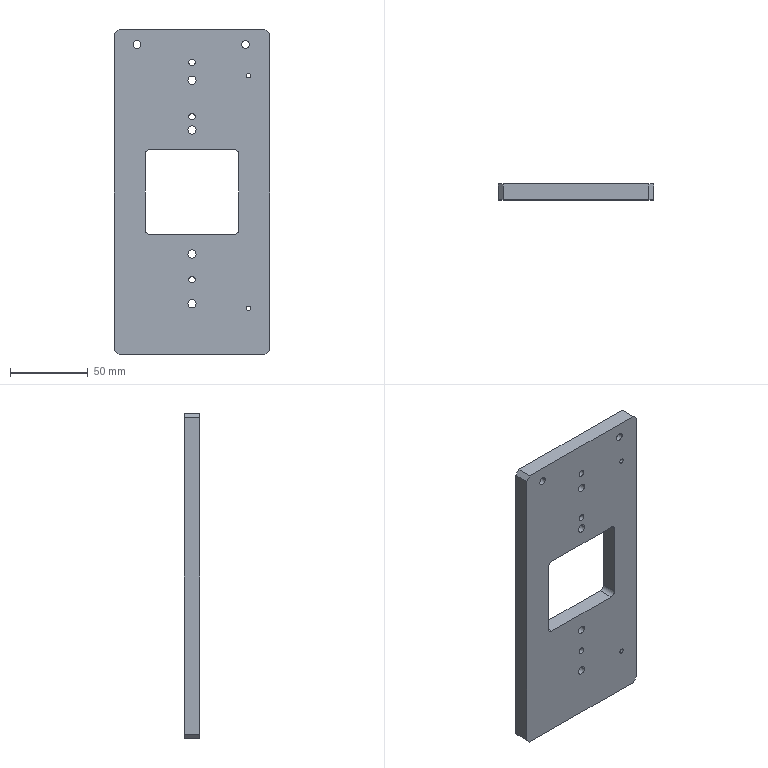Component | SolidWorks | SFTJ-06-CylinderBackPlate-1 | 1 solid | 60 faces | box 100 x 10 x 210 mm | volume 173599 mm3 | cylinder 38 | plane 18 | cone 4 | commonest cylinder face diameters 10 x8 5.3 x8 4.2 x6 5 x4 3.3 x4 3 x4 6 x4 | material 6061 Alloy
build123d program:
from build123d import *

# Parameters (mm, degrees)
SKETCH1_W                                            = 100
SKETCH1_H                                            = 210
BOSS_EXTRUDE1_DEPTH                                  = 5
CHAMFER1_SIZE                                        = 3
SKETCH2_W                                            = 60
SKETCH2_H                                            = 55
CUT_EXTRUDE1_DEPTH                                   = 117.726
FILLET1_R                                            = 3
M5_TAPPED_HOLE1_D                                    = 4.2
HOLE_SIZE_ACCORDING_TO_HEX_SOCKET_HEAD_C_D           = 5.3
HOLE_SIZE_ACCORDING_TO_HEX_SOCKET_HEAD_C_CBORE_D     = 10
HOLE_SIZE_ACCORDING_TO_HEX_SOCKET_HEAD_C_CBORE_DEPTH = 5.7
SIZE_MM_DOWEL_PIN_HOLE2_D                            = 3
M4_TAPPED_HOLE1_D                                    = 3.3
M4_TAPPED_HOLE1_DEPTH                                = 10.1
M4_TAPPED_HOLE1_TIP                                  = 0.9914
M6_TAPPED_HOLE1_D                                    = 5


with BuildPart() as part:
    # Sketch1 → Boss-Extrude1 (new, symmetric)
    with BuildSketch(Plane.XY):
        Rectangle(SKETCH1_W, SKETCH1_H)
    extrude(amount=BOSS_EXTRUDE1_DEPTH, both=True)

    # Chamfer1
    chamfer1_edges = [part.edges().sort_by_distance(p)[0] for p in [
        (-50, 105, 0),
        (50, 105, 0),
        (50, -105, 0),
        (-50, -105, 0),
    ]]
    chamfer(chamfer1_edges, length=CHAMFER1_SIZE)

    # Sketch2 → Cut-Extrude1 (cut, through all)
    with BuildSketch(Plane(origin=(0, 0, -5), x_dir=(-1, 0, 0), z_dir=(0, 0, -1))):
        Rectangle(SKETCH2_W, SKETCH2_H)
    extrude(amount=-CUT_EXTRUDE1_DEPTH, mode=Mode.SUBTRACT)

    # Fillet1
    fillet1_edges = [part.edges().sort_by_distance(p)[0] for p in [
        (30, -27.5, 0),
        (30, 27.5, 0),
        (-30, 27.5, 0),
        (-30, -27.5, 0),
    ]]
    fillet(fillet1_edges, radius=FILLET1_R)

    # M5 Tapped Hole1 (through all)
    with Locations(Plane(origin=(0, 0, -5), x_dir=(-1, 0, 0), z_dir=(0, 0, -1))):
        with Locations((0, -56.5), (0, 48.5), (0, 83.5)):
            Hole(M5_TAPPED_HOLE1_D / 2)

    # Hole Size according to Hex Socket Head C (through all)
    with Locations(Plane(origin=(0, 0, -5), x_dir=(-1, 0, 0), z_dir=(0, 0, -1))):
        with Locations((0, -72), (0, -40), (0, 40), (0, 72)):
            CounterBoreHole(HOLE_SIZE_ACCORDING_TO_HEX_SOCKET_HEAD_C_D / 2, HOLE_SIZE_ACCORDING_TO_HEX_SOCKET_HEAD_C_CBORE_D / 2, HOLE_SIZE_ACCORDING_TO_HEX_SOCKET_HEAD_C_CBORE_DEPTH)

    # Size mm Dowel Pin Hole2 (through all)
    with Locations(Plane(origin=(0, 0, -5), x_dir=(-1, 0, 0), z_dir=(0, 0, -1))):
        with Locations((-36.5, -75), (-36.5, 75)):
            Hole(SIZE_MM_DOWEL_PIN_HOLE2_D / 2)

    # M4 Tapped Hole1
    with Locations(Plane(origin=(0, -105, 0), x_dir=(-1, 0, 0), z_dir=(0, -1, 0))):
        with Locations((-7.5, 1), (7.5, 1)):
            Hole(M4_TAPPED_HOLE1_D / 2, depth=M4_TAPPED_HOLE1_DEPTH)
            with Locations((0, 0, -(M4_TAPPED_HOLE1_DEPTH + M4_TAPPED_HOLE1_TIP / 2))):  # 118° drill point
                Cone(0, M4_TAPPED_HOLE1_D / 2, M4_TAPPED_HOLE1_TIP, mode=Mode.SUBTRACT)

    # M6 Tapped Hole1 (through all)
    with Locations(Plane.XY.offset(5)):
        with Locations((34.5, 95), (-35.5, 95)):
            Hole(M6_TAPPED_HOLE1_D / 2)


solid = part.part

# Placed as in the assembly
solid = solid.moved(Location((-235.009, 45.721, 38.589), (90, 0, 0)))